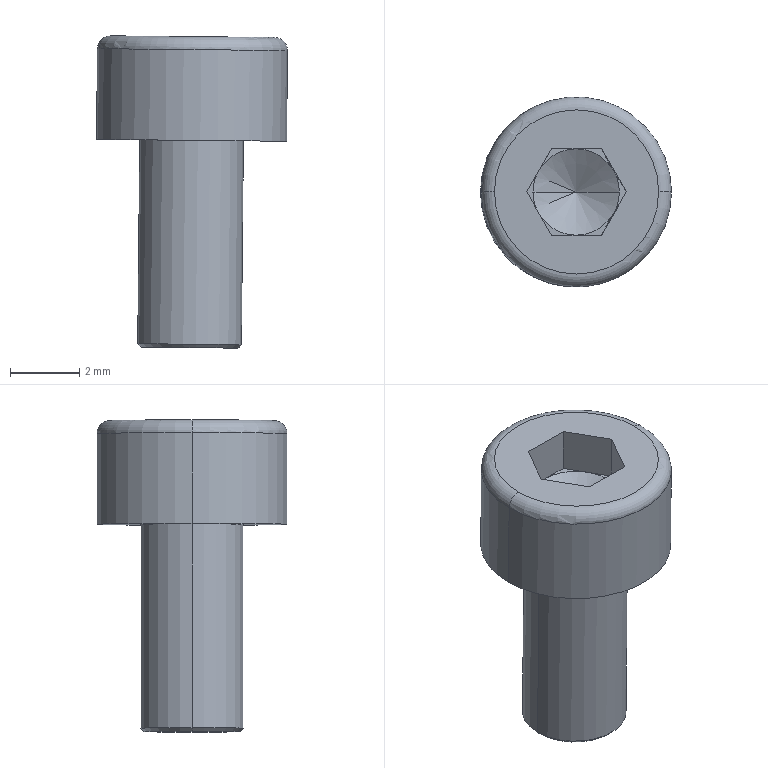Component | SolidWorks | hexagon socket head cap screws gb-20 | 1 solid | 25 faces | box 5.53 x 5.5 x 9.04 mm | volume 105 mm3 | plane 15 | cone 4 | cylinder 4 | torus 2 | commonest cylinder face diameters 3 x2 5.5 x2
STEP:
#1=CARTESIAN_POINT('',(-0.2262,1.201,0.7367));
#2=VERTEX_POINT('',#1);
#3=CARTESIAN_POINT('',(-0.116,1.201,0.7356));
#4=VERTEX_POINT('',#3);
#5=CARTESIAN_POINT('',(-0.1711,1.201,0.7361));
#6=DIRECTION('',(-0.009793,-0.,-1.));
#7=DIRECTION('',(-1.,0.,0.009793));
#8=AXIS2_PLACEMENT_3D('',#5,#6,#7);
#9=CIRCLE('',#8,0.05512);
#10=EDGE_CURVE('',#2,#4,#9,.T.);
#11=ORIENTED_EDGE('',*,*,#10,.F.);
#12=CARTESIAN_POINT('',(-0.2301,1.201,0.7406));
#13=VERTEX_POINT('',#12);
#14=CARTESIAN_POINT('',(-0.2262,1.201,0.7367));
#15=DIRECTION('',(-0.7001,-0.,0.714));
#16=VECTOR('',#15,39.37);
#17=LINE('',#14,#16);
#18=EDGE_CURVE('',#2,#13,#17,.T.);
#19=ORIENTED_EDGE('',*,*,#18,.T.);
#20=CARTESIAN_POINT('',(-0.112,1.201,0.7395));
#21=VERTEX_POINT('',#20);
#22=CARTESIAN_POINT('',(-0.1711,1.201,0.7401));
#23=DIRECTION('',(0.009793,0.,1.));
#24=DIRECTION('',(-1.,-0.,0.009793));
#25=AXIS2_PLACEMENT_3D('',#22,#23,#24);
#26=CIRCLE('',#25,0.05906);
#27=EDGE_CURVE('',#21,#13,#26,.T.);
#28=ORIENTED_EDGE('',*,*,#27,.F.);
#29=CARTESIAN_POINT('',(-0.116,1.201,0.7356));
#30=DIRECTION('',(0.714,0.,0.7001));
#31=VECTOR('',#30,39.37);
#32=LINE('',#29,#31);
#33=EDGE_CURVE('',#4,#21,#32,.T.);
#34=ORIENTED_EDGE('',*,*,#33,.F.);
#35=EDGE_LOOP('',(#11,#19,#28,#34));
#36=FACE_OUTER_BOUND('',#35,.T.);
#37=CARTESIAN_POINT('',(-0.1711,1.201,0.7361));
#38=DIRECTION('',(0.009793,0.,1.));
#39=DIRECTION('',(1.,0.,-0.009793));
#40=AXIS2_PLACEMENT_3D('',#37,#38,#39);
#41=CONICAL_SURFACE('',#40,0.05512,0.7854);
#42=ADVANCED_FACE('',(#36),#41,.T.);
#43=CARTESIAN_POINT('',(-0.07416,1.201,1.09));
#44=VERTEX_POINT('',#43);
#45=CARTESIAN_POINT('',(-0.2612,1.201,1.091));
#46=VERTEX_POINT('',#45);
#47=CARTESIAN_POINT('',(-0.1677,1.201,1.09));
#48=DIRECTION('',(0.009793,0.,1.));
#49=DIRECTION('',(-1.,-0.,0.009793));
#50=AXIS2_PLACEMENT_3D('',#47,#48,#49);
#51=CIRCLE('',#50,0.0935);
#52=EDGE_CURVE('',#44,#46,#51,.T.);
#53=ORIENTED_EDGE('',*,*,#52,.F.);
#54=CARTESIAN_POINT('',(-0.05955,1.201,1.075));
#55=VERTEX_POINT('',#54);
#56=CARTESIAN_POINT('',(-0.07431,1.201,1.075));
#57=DIRECTION('',(-0.,1.,-0.));
#58=DIRECTION('',(-1.,0.,0.));
#59=AXIS2_PLACEMENT_3D('',#56,#57,#58);
#60=CIRCLE('',#59,0.01476);
#61=EDGE_CURVE('',#44,#55,#60,.T.);
#62=ORIENTED_EDGE('',*,*,#61,.T.);
#63=CARTESIAN_POINT('',(-0.2761,1.201,1.077));
#64=VERTEX_POINT('',#63);
#65=CARTESIAN_POINT('',(-0.1678,1.201,1.076));
#66=DIRECTION('',(-0.009793,-0.,-1.));
#67=DIRECTION('',(-1.,-0.,0.009793));
#68=AXIS2_PLACEMENT_3D('',#65,#66,#67);
#69=CIRCLE('',#68,0.1083);
#70=EDGE_CURVE('',#64,#55,#69,.T.);
#71=ORIENTED_EDGE('',*,*,#70,.F.);
#72=CARTESIAN_POINT('',(-0.2613,1.201,1.077));
#73=DIRECTION('',(0.,-1.,0.));
#74=DIRECTION('',(1.,0.,0.));
#75=AXIS2_PLACEMENT_3D('',#72,#73,#74);
#76=CIRCLE('',#75,0.01476);
#77=EDGE_CURVE('',#46,#64,#76,.T.);
#78=ORIENTED_EDGE('',*,*,#77,.F.);
#79=EDGE_LOOP('',(#53,#62,#71,#78));
#80=FACE_OUTER_BOUND('',#79,.T.);
#81=CARTESIAN_POINT('',(-0.1678,1.201,1.076));
#82=DIRECTION('',(-0.009793,-0.,-1.));
#83=DIRECTION('',(-1.,-0.,0.009793));
#84=AXIS2_PLACEMENT_3D('',#81,#82,#83);
#85=TOROIDAL_SURFACE('',#84,0.0935,0.01476);
#86=ADVANCED_FACE('',(#80),#85,.T.);
#87=CARTESIAN_POINT('',(-0.1684,1.201,1.011));
#88=VERTEX_POINT('',#87);
#89=CARTESIAN_POINT('',(-0.119,1.201,1.039));
#90=VERTEX_POINT('',#89);
#91=CARTESIAN_POINT('',(-0.119,1.201,1.039));
#92=DIRECTION('',(0.8709,0.,0.4915));
#93=VECTOR('',#92,39.37);
#94=LINE('',#91,#93);
#95=EDGE_CURVE('',#88,#90,#94,.T.);
#96=ORIENTED_EDGE('',*,*,#95,.F.);
#97=CARTESIAN_POINT('',(-0.2174,1.201,1.04));
#98=VERTEX_POINT('',#97);
#99=CARTESIAN_POINT('',(-0.2174,1.201,1.04));
#100=DIRECTION('',(-0.8611,-0.,0.5085));
#101=VECTOR('',#100,39.37);
#102=LINE('',#99,#101);
#103=EDGE_CURVE('',#88,#98,#102,.T.);
#104=ORIENTED_EDGE('',*,*,#103,.T.);
#105=CARTESIAN_POINT('',(-0.2108,1.176,1.04));
#106=VERTEX_POINT('',#105);
#107=CARTESIAN_POINT('',(-0.1682,1.201,1.039));
#108=DIRECTION('',(-0.009793,-0.,-1.));
#109=DIRECTION('',(1.,0.,-0.009793));
#110=AXIS2_PLACEMENT_3D('',#107,#108,#109);
#111=CIRCLE('',#110,0.04921);
#112=EDGE_CURVE('',#106,#98,#111,.T.);
#113=ORIENTED_EDGE('',*,*,#112,.F.);
#114=CARTESIAN_POINT('',(-0.1682,1.151,1.039));
#115=VERTEX_POINT('',#114);
#116=CARTESIAN_POINT('',(-0.1682,1.201,1.039));
#117=DIRECTION('',(-0.009793,-0.,-1.));
#118=DIRECTION('',(1.,0.,-0.009793));
#119=AXIS2_PLACEMENT_3D('',#116,#117,#118);
#120=CIRCLE('',#119,0.04921);
#121=EDGE_CURVE('',#115,#106,#120,.T.);
#122=ORIENTED_EDGE('',*,*,#121,.F.);
#123=CARTESIAN_POINT('',(-0.1255,1.176,1.039));
#124=VERTEX_POINT('',#123);
#125=CARTESIAN_POINT('',(-0.1682,1.201,1.039));
#126=DIRECTION('',(-0.009793,-0.,-1.));
#127=DIRECTION('',(1.,0.,-0.009793));
#128=AXIS2_PLACEMENT_3D('',#125,#126,#127);
#129=CIRCLE('',#128,0.04921);
#130=EDGE_CURVE('',#124,#115,#129,.T.);
#131=ORIENTED_EDGE('',*,*,#130,.F.);
#132=CARTESIAN_POINT('',(-0.1682,1.201,1.039));
#133=DIRECTION('',(-0.009793,-0.,-1.));
#134=DIRECTION('',(1.,0.,-0.009793));
#135=AXIS2_PLACEMENT_3D('',#132,#133,#134);
#136=CIRCLE('',#135,0.04921);
#137=EDGE_CURVE('',#90,#124,#136,.T.);
#138=ORIENTED_EDGE('',*,*,#137,.F.);
#139=EDGE_LOOP('',(#96,#104,#113,#122,#131,#138));
#140=FACE_OUTER_BOUND('',#139,.T.);
#141=CARTESIAN_POINT('',(-0.1682,1.201,1.039));
#142=DIRECTION('',(0.009793,0.,1.));
#143=DIRECTION('',(1.,0.,-0.009793));
#144=AXIS2_PLACEMENT_3D('',#141,#142,#143);
#145=CONICAL_SURFACE('',#144,0.04921,1.047);
#146=ADVANCED_FACE('',(#140),#145,.F.);
#147=ORIENTED_EDGE('',*,*,#27,.T.);
#148=CARTESIAN_POINT('',(-0.2279,1.201,0.9729));
#149=VERTEX_POINT('',#148);
#150=CARTESIAN_POINT('',(-0.2302,1.201,0.7367));
#151=DIRECTION('',(0.009793,0.,1.));
#152=VECTOR('',#151,39.37);
#153=LINE('',#150,#152);
#154=EDGE_CURVE('',#13,#149,#153,.T.);
#155=ORIENTED_EDGE('',*,*,#154,.T.);
#156=CARTESIAN_POINT('',(-0.1098,1.201,0.9718));
#157=VERTEX_POINT('',#156);
#158=CARTESIAN_POINT('',(-0.1688,1.201,0.9723));
#159=DIRECTION('',(-0.009793,-0.,-1.));
#160=DIRECTION('',(-1.,0.,0.009793));
#161=AXIS2_PLACEMENT_3D('',#158,#159,#160);
#162=CIRCLE('',#161,0.05906);
#163=EDGE_CURVE('',#149,#157,#162,.T.);
#164=ORIENTED_EDGE('',*,*,#163,.T.);
#165=CARTESIAN_POINT('',(-0.1121,1.201,0.7355));
#166=DIRECTION('',(0.009793,0.,1.));
#167=VECTOR('',#166,39.37);
#168=LINE('',#165,#167);
#169=EDGE_CURVE('',#21,#157,#168,.T.);
#170=ORIENTED_EDGE('',*,*,#169,.F.);
#171=EDGE_LOOP('',(#147,#155,#164,#170));
#172=FACE_OUTER_BOUND('',#171,.T.);
#173=CARTESIAN_POINT('',(-0.1711,1.201,0.7361));
#174=DIRECTION('',(0.009793,0.,1.));
#175=DIRECTION('',(1.,0.,-0.009793));
#176=AXIS2_PLACEMENT_3D('',#173,#174,#175);
#177=CYLINDRICAL_SURFACE('',#176,0.05906);
#178=ADVANCED_FACE('',(#172),#177,.T.);
#179=CARTESIAN_POINT('',(-0.2771,1.201,0.9734));
#180=VERTEX_POINT('',#179);
#181=CARTESIAN_POINT('',(-0.06056,1.201,0.9713));
#182=VERTEX_POINT('',#181);
#183=CARTESIAN_POINT('',(-0.1688,1.201,0.9723));
#184=DIRECTION('',(-0.009793,-0.,-1.));
#185=DIRECTION('',(-1.,-0.,0.009793));
#186=AXIS2_PLACEMENT_3D('',#183,#184,#185);
#187=CIRCLE('',#186,0.1083);
#188=EDGE_CURVE('',#180,#182,#187,.T.);
#189=ORIENTED_EDGE('',*,*,#188,.F.);
#190=CARTESIAN_POINT('',(-0.2771,1.201,0.9734));
#191=DIRECTION('',(0.009793,0.,1.));
#192=VECTOR('',#191,39.37);
#193=LINE('',#190,#192);
#194=EDGE_CURVE('',#180,#64,#193,.T.);
#195=ORIENTED_EDGE('',*,*,#194,.T.);
#196=ORIENTED_EDGE('',*,*,#70,.T.);
#197=CARTESIAN_POINT('',(-0.06056,1.201,0.9713));
#198=DIRECTION('',(0.009793,0.,1.));
#199=VECTOR('',#198,39.37);
#200=LINE('',#197,#199);
#201=EDGE_CURVE('',#182,#55,#200,.T.);
#202=ORIENTED_EDGE('',*,*,#201,.F.);
#203=EDGE_LOOP('',(#189,#195,#196,#202));
#204=FACE_OUTER_BOUND('',#203,.T.);
#205=CARTESIAN_POINT('',(-0.1688,1.201,0.9723));
#206=DIRECTION('',(0.009793,0.,1.));
#207=DIRECTION('',(1.,0.,-0.009793));
#208=AXIS2_PLACEMENT_3D('',#205,#206,#207);
#209=CYLINDRICAL_SURFACE('',#208,0.1083);
#210=ADVANCED_FACE('',(#204),#209,.T.);
#211=CARTESIAN_POINT('',(-0.1398,1.151,1.039));
#212=VERTEX_POINT('',#211);
#213=CARTESIAN_POINT('',(-0.1113,1.201,1.039));
#214=DIRECTION('',(-0.5,-0.866,0.004897));
#215=VECTOR('',#214,39.37);
#216=LINE('',#213,#215);
#217=EDGE_CURVE('',#124,#212,#216,.T.);
#218=ORIENTED_EDGE('',*,*,#217,.F.);
#219=ORIENTED_EDGE('',*,*,#130,.T.);
#220=CARTESIAN_POINT('',(-0.1398,1.151,1.039));
#221=DIRECTION('',(-1.,-0.,0.009793));
#222=VECTOR('',#221,39.37);
#223=LINE('',#220,#222);
#224=EDGE_CURVE('',#212,#115,#223,.T.);
#225=ORIENTED_EDGE('',*,*,#224,.F.);
#226=EDGE_LOOP('',(#218,#219,#225));
#227=FACE_OUTER_BOUND('',#226,.T.);
#228=CARTESIAN_POINT('',(-0.1682,1.102,1.039));
#229=DIRECTION('',(0.009793,0.,1.));
#230=DIRECTION('',(1.,0.,-0.009793));
#231=AXIS2_PLACEMENT_3D('',#228,#229,#230);
#232=PLANE('',#231);
#233=ADVANCED_FACE('',(#227),#232,.T.);
#234=CARTESIAN_POINT('',(-0.1966,1.151,1.04));
#235=VERTEX_POINT('',#234);
#236=CARTESIAN_POINT('',(-0.1398,1.151,1.039));
#237=DIRECTION('',(-1.,-0.,0.009793));
#238=VECTOR('',#237,39.37);
#239=LINE('',#236,#238);
#240=EDGE_CURVE('',#115,#235,#239,.T.);
#241=ORIENTED_EDGE('',*,*,#240,.F.);
#242=ORIENTED_EDGE('',*,*,#121,.T.);
#243=CARTESIAN_POINT('',(-0.1966,1.151,1.04));
#244=DIRECTION('',(-0.5,0.866,0.004897));
#245=VECTOR('',#244,39.37);
#246=LINE('',#243,#245);
#247=EDGE_CURVE('',#235,#106,#246,.T.);
#248=ORIENTED_EDGE('',*,*,#247,.F.);
#249=EDGE_LOOP('',(#241,#242,#248));
#250=FACE_OUTER_BOUND('',#249,.T.);
#251=CARTESIAN_POINT('',(-0.1682,1.102,1.039));
#252=DIRECTION('',(0.009793,0.,1.));
#253=DIRECTION('',(1.,0.,-0.009793));
#254=AXIS2_PLACEMENT_3D('',#251,#252,#253);
#255=PLANE('',#254);
#256=ADVANCED_FACE('',(#250),#255,.T.);
#257=CARTESIAN_POINT('',(-0.225,1.201,1.04));
#258=VERTEX_POINT('',#257);
#259=CARTESIAN_POINT('',(-0.1966,1.151,1.04));
#260=DIRECTION('',(-0.5,0.866,0.004897));
#261=VECTOR('',#260,39.37);
#262=LINE('',#259,#261);
#263=EDGE_CURVE('',#106,#258,#262,.T.);
#264=ORIENTED_EDGE('',*,*,#263,.F.);
#265=ORIENTED_EDGE('',*,*,#112,.T.);
#266=CARTESIAN_POINT('',(-0.2108,1.225,1.04));
#267=VERTEX_POINT('',#266);
#268=CARTESIAN_POINT('',(-0.1682,1.201,1.039));
#269=DIRECTION('',(-0.009793,-0.,-1.));
#270=DIRECTION('',(1.,-0.,-0.009793));
#271=AXIS2_PLACEMENT_3D('',#268,#269,#270);
#272=CIRCLE('',#271,0.04921);
#273=EDGE_CURVE('',#98,#267,#272,.T.);
#274=ORIENTED_EDGE('',*,*,#273,.T.);
#275=CARTESIAN_POINT('',(-0.225,1.201,1.04));
#276=DIRECTION('',(0.5,0.866,-0.004897));
#277=VECTOR('',#276,39.37);
#278=LINE('',#275,#277);
#279=EDGE_CURVE('',#258,#267,#278,.T.);
#280=ORIENTED_EDGE('',*,*,#279,.F.);
#281=EDGE_LOOP('',(#264,#265,#274,#280));
#282=FACE_OUTER_BOUND('',#281,.T.);
#283=CARTESIAN_POINT('',(-0.1682,1.102,1.039));
#284=DIRECTION('',(0.009793,0.,1.));
#285=DIRECTION('',(1.,0.,-0.009793));
#286=AXIS2_PLACEMENT_3D('',#283,#284,#285);
#287=PLANE('',#286);
#288=ADVANCED_FACE('',(#282),#287,.T.);
#289=CARTESIAN_POINT('',(-0.1966,1.25,1.04));
#290=VERTEX_POINT('',#289);
#291=CARTESIAN_POINT('',(-0.225,1.201,1.04));
#292=DIRECTION('',(0.5,0.866,-0.004897));
#293=VECTOR('',#292,39.37);
#294=LINE('',#291,#293);
#295=EDGE_CURVE('',#267,#290,#294,.T.);
#296=ORIENTED_EDGE('',*,*,#295,.F.);
#297=CARTESIAN_POINT('',(-0.1682,1.25,1.039));
#298=VERTEX_POINT('',#297);
#299=CARTESIAN_POINT('',(-0.1682,1.201,1.039));
#300=DIRECTION('',(-0.009793,-0.,-1.));
#301=DIRECTION('',(-1.,0.,0.009793));
#302=AXIS2_PLACEMENT_3D('',#299,#300,#301);
#303=CIRCLE('',#302,0.04921);
#304=EDGE_CURVE('',#267,#298,#303,.T.);
#305=ORIENTED_EDGE('',*,*,#304,.T.);
#306=CARTESIAN_POINT('',(-0.1966,1.25,1.04));
#307=DIRECTION('',(1.,0.,-0.009793));
#308=VECTOR('',#307,39.37);
#309=LINE('',#306,#308);
#310=EDGE_CURVE('',#290,#298,#309,.T.);
#311=ORIENTED_EDGE('',*,*,#310,.F.);
#312=EDGE_LOOP('',(#296,#305,#311));
#313=FACE_OUTER_BOUND('',#312,.T.);
#314=CARTESIAN_POINT('',(-0.1682,1.102,1.039));
#315=DIRECTION('',(0.009793,0.,1.));
#316=DIRECTION('',(1.,0.,-0.009793));
#317=AXIS2_PLACEMENT_3D('',#314,#315,#316);
#318=PLANE('',#317);
#319=ADVANCED_FACE('',(#313),#318,.T.);
#320=CARTESIAN_POINT('',(-0.1398,1.25,1.039));
#321=VERTEX_POINT('',#320);
#322=CARTESIAN_POINT('',(-0.1966,1.25,1.04));
#323=DIRECTION('',(1.,0.,-0.009793));
#324=VECTOR('',#323,39.37);
#325=LINE('',#322,#324);
#326=EDGE_CURVE('',#298,#321,#325,.T.);
#327=ORIENTED_EDGE('',*,*,#326,.F.);
#328=CARTESIAN_POINT('',(-0.1255,1.225,1.039));
#329=VERTEX_POINT('',#328);
#330=CARTESIAN_POINT('',(-0.1682,1.201,1.039));
#331=DIRECTION('',(-0.009793,-0.,-1.));
#332=DIRECTION('',(1.,0.,-0.009793));
#333=AXIS2_PLACEMENT_3D('',#330,#331,#332);
#334=CIRCLE('',#333,0.04921);
#335=EDGE_CURVE('',#298,#329,#334,.T.);
#336=ORIENTED_EDGE('',*,*,#335,.T.);
#337=CARTESIAN_POINT('',(-0.1398,1.25,1.039));
#338=DIRECTION('',(0.5,-0.866,-0.004897));
#339=VECTOR('',#338,39.37);
#340=LINE('',#337,#339);
#341=EDGE_CURVE('',#321,#329,#340,.T.);
#342=ORIENTED_EDGE('',*,*,#341,.F.);
#343=EDGE_LOOP('',(#327,#336,#342));
#344=FACE_OUTER_BOUND('',#343,.T.);
#345=CARTESIAN_POINT('',(-0.1682,1.102,1.039));
#346=DIRECTION('',(0.009793,0.,1.));
#347=DIRECTION('',(1.,0.,-0.009793));
#348=AXIS2_PLACEMENT_3D('',#345,#346,#347);
#349=PLANE('',#348);
#350=ADVANCED_FACE('',(#344),#349,.T.);
#351=CARTESIAN_POINT('',(-0.1113,1.201,1.039));
#352=VERTEX_POINT('',#351);
#353=CARTESIAN_POINT('',(-0.1398,1.25,1.039));
#354=DIRECTION('',(0.5,-0.866,-0.004897));
#355=VECTOR('',#354,39.37);
#356=LINE('',#353,#355);
#357=EDGE_CURVE('',#329,#352,#356,.T.);
#358=ORIENTED_EDGE('',*,*,#357,.F.);
#359=CARTESIAN_POINT('',(-0.1682,1.201,1.039));
#360=DIRECTION('',(-0.009793,-0.,-1.));
#361=DIRECTION('',(1.,0.,-0.009793));
#362=AXIS2_PLACEMENT_3D('',#359,#360,#361);
#363=CIRCLE('',#362,0.04921);
#364=EDGE_CURVE('',#329,#90,#363,.T.);
#365=ORIENTED_EDGE('',*,*,#364,.T.);
#366=ORIENTED_EDGE('',*,*,#137,.T.);
#367=CARTESIAN_POINT('',(-0.1113,1.201,1.039));
#368=DIRECTION('',(-0.5,-0.866,0.004897));
#369=VECTOR('',#368,39.37);
#370=LINE('',#367,#369);
#371=EDGE_CURVE('',#352,#124,#370,.T.);
#372=ORIENTED_EDGE('',*,*,#371,.F.);
#373=EDGE_LOOP('',(#358,#365,#366,#372));
#374=FACE_OUTER_BOUND('',#373,.T.);
#375=CARTESIAN_POINT('',(-0.1682,1.102,1.039));
#376=DIRECTION('',(0.009793,0.,1.));
#377=DIRECTION('',(1.,0.,-0.009793));
#378=AXIS2_PLACEMENT_3D('',#375,#376,#377);
#379=PLANE('',#378);
#380=ADVANCED_FACE('',(#374),#379,.T.);
#381=CARTESIAN_POINT('',(-0.1677,1.201,1.09));
#382=DIRECTION('',(0.009793,0.,1.));
#383=DIRECTION('',(-1.,-0.,0.009793));
#384=AXIS2_PLACEMENT_3D('',#381,#382,#383);
#385=CIRCLE('',#384,0.0935);
#386=EDGE_CURVE('',#46,#44,#385,.T.);
#387=ORIENTED_EDGE('',*,*,#386,.T.);
#388=ORIENTED_EDGE('',*,*,#52,.T.);
#389=EDGE_LOOP('',(#387,#388));
#390=FACE_OUTER_BOUND('',#389,.T.);
#391=CARTESIAN_POINT('',(-0.1961,1.151,1.091));
#392=VERTEX_POINT('',#391);
#393=CARTESIAN_POINT('',(-0.2245,1.201,1.091));
#394=VERTEX_POINT('',#393);
#395=CARTESIAN_POINT('',(-0.1961,1.151,1.091));
#396=DIRECTION('',(-0.5,0.866,0.004897));
#397=VECTOR('',#396,39.37);
#398=LINE('',#395,#397);
#399=EDGE_CURVE('',#392,#394,#398,.T.);
#400=ORIENTED_EDGE('',*,*,#399,.T.);
#401=CARTESIAN_POINT('',(-0.1961,1.25,1.091));
#402=VERTEX_POINT('',#401);
#403=CARTESIAN_POINT('',(-0.2245,1.201,1.091));
#404=DIRECTION('',(0.5,0.866,-0.004897));
#405=VECTOR('',#404,39.37);
#406=LINE('',#403,#405);
#407=EDGE_CURVE('',#394,#402,#406,.T.);
#408=ORIENTED_EDGE('',*,*,#407,.T.);
#409=CARTESIAN_POINT('',(-0.1393,1.25,1.09));
#410=VERTEX_POINT('',#409);
#411=CARTESIAN_POINT('',(-0.1961,1.25,1.091));
#412=DIRECTION('',(1.,0.,-0.009793));
#413=VECTOR('',#412,39.37);
#414=LINE('',#411,#413);
#415=EDGE_CURVE('',#402,#410,#414,.T.);
#416=ORIENTED_EDGE('',*,*,#415,.T.);
#417=CARTESIAN_POINT('',(-0.1108,1.201,1.09));
#418=VERTEX_POINT('',#417);
#419=CARTESIAN_POINT('',(-0.1393,1.25,1.09));
#420=DIRECTION('',(0.5,-0.866,-0.004897));
#421=VECTOR('',#420,39.37);
#422=LINE('',#419,#421);
#423=EDGE_CURVE('',#410,#418,#422,.T.);
#424=ORIENTED_EDGE('',*,*,#423,.T.);
#425=CARTESIAN_POINT('',(-0.1393,1.151,1.09));
#426=VERTEX_POINT('',#425);
#427=CARTESIAN_POINT('',(-0.1108,1.201,1.09));
#428=DIRECTION('',(-0.5,-0.866,0.004897));
#429=VECTOR('',#428,39.37);
#430=LINE('',#427,#429);
#431=EDGE_CURVE('',#418,#426,#430,.T.);
#432=ORIENTED_EDGE('',*,*,#431,.T.);
#433=CARTESIAN_POINT('',(-0.1393,1.151,1.09));
#434=DIRECTION('',(-1.,-0.,0.009793));
#435=VECTOR('',#434,39.37);
#436=LINE('',#433,#435);
#437=EDGE_CURVE('',#426,#392,#436,.T.);
#438=ORIENTED_EDGE('',*,*,#437,.T.);
#439=EDGE_LOOP('',(#400,#408,#416,#424,#432,#438));
#440=FACE_BOUND('',#439,.T.);
#441=CARTESIAN_POINT('',(-0.1677,1.201,1.09));
#442=DIRECTION('',(-0.009793,-0.,-1.));
#443=DIRECTION('',(-1.,-0.,0.009793));
#444=AXIS2_PLACEMENT_3D('',#441,#442,#443);
#445=PLANE('',#444);
#446=ADVANCED_FACE('',(#390,#440),#445,.F.);
#447=CARTESIAN_POINT('',(-0.1688,1.201,0.9723));
#448=DIRECTION('',(-0.009793,-0.,-1.));
#449=DIRECTION('',(-1.,-0.,0.009793));
#450=AXIS2_PLACEMENT_3D('',#447,#448,#449);
#451=CIRCLE('',#450,0.1083);
#452=EDGE_CURVE('',#182,#180,#451,.T.);
#453=ORIENTED_EDGE('',*,*,#452,.T.);
#454=ORIENTED_EDGE('',*,*,#188,.T.);
#455=EDGE_LOOP('',(#453,#454));
#456=FACE_OUTER_BOUND('',#455,.T.);
#457=CARTESIAN_POINT('',(-0.1688,1.201,0.9723));
#458=DIRECTION('',(-0.009793,-0.,-1.));
#459=DIRECTION('',(-1.,0.,0.009793));
#460=AXIS2_PLACEMENT_3D('',#457,#458,#459);
#461=CIRCLE('',#460,0.05906);
#462=EDGE_CURVE('',#157,#149,#461,.T.);
#463=ORIENTED_EDGE('',*,*,#462,.F.);
#464=ORIENTED_EDGE('',*,*,#163,.F.);
#465=EDGE_LOOP('',(#463,#464));
#466=FACE_BOUND('',#465,.T.);
#467=CARTESIAN_POINT('',(-0.1688,1.201,0.9723));
#468=DIRECTION('',(-0.009793,-0.,-1.));
#469=DIRECTION('',(-1.,-0.,0.009793));
#470=AXIS2_PLACEMENT_3D('',#467,#468,#469);
#471=PLANE('',#470);
#472=ADVANCED_FACE('',(#456,#466),#471,.T.);
#473=ORIENTED_EDGE('',*,*,#194,.F.);
#474=ORIENTED_EDGE('',*,*,#452,.F.);
#475=ORIENTED_EDGE('',*,*,#201,.T.);
#476=CARTESIAN_POINT('',(-0.1678,1.201,1.076));
#477=DIRECTION('',(-0.009793,-0.,-1.));
#478=DIRECTION('',(-1.,-0.,0.009793));
#479=AXIS2_PLACEMENT_3D('',#476,#477,#478);
#480=CIRCLE('',#479,0.1083);
#481=EDGE_CURVE('',#55,#64,#480,.T.);
#482=ORIENTED_EDGE('',*,*,#481,.T.);
#483=EDGE_LOOP('',(#473,#474,#475,#482));
#484=FACE_OUTER_BOUND('',#483,.T.);
#485=CARTESIAN_POINT('',(-0.1688,1.201,0.9723));
#486=DIRECTION('',(0.009793,0.,1.));
#487=DIRECTION('',(1.,0.,-0.009793));
#488=AXIS2_PLACEMENT_3D('',#485,#486,#487);
#489=CYLINDRICAL_SURFACE('',#488,0.1083);
#490=ADVANCED_FACE('',(#484),#489,.T.);
#491=ORIENTED_EDGE('',*,*,#154,.F.);
#492=CARTESIAN_POINT('',(-0.1711,1.201,0.7401));
#493=DIRECTION('',(0.009793,0.,1.));
#494=DIRECTION('',(-1.,-0.,0.009793));
#495=AXIS2_PLACEMENT_3D('',#492,#493,#494);
#496=CIRCLE('',#495,0.05906);
#497=EDGE_CURVE('',#13,#21,#496,.T.);
#498=ORIENTED_EDGE('',*,*,#497,.T.);
#499=ORIENTED_EDGE('',*,*,#169,.T.);
#500=ORIENTED_EDGE('',*,*,#462,.T.);
#501=EDGE_LOOP('',(#491,#498,#499,#500));
#502=FACE_OUTER_BOUND('',#501,.T.);
#503=CARTESIAN_POINT('',(-0.1711,1.201,0.7361));
#504=DIRECTION('',(0.009793,0.,1.));
#505=DIRECTION('',(1.,0.,-0.009793));
#506=AXIS2_PLACEMENT_3D('',#503,#504,#505);
#507=CYLINDRICAL_SURFACE('',#506,0.05906);
#508=ADVANCED_FACE('',(#502),#507,.T.);
#509=CARTESIAN_POINT('',(-0.1711,1.201,0.7361));
#510=DIRECTION('',(-0.009793,-0.,-1.));
#511=DIRECTION('',(-1.,0.,0.009793));
#512=AXIS2_PLACEMENT_3D('',#509,#510,#511);
#513=CIRCLE('',#512,0.05512);
#514=EDGE_CURVE('',#4,#2,#513,.T.);
#515=ORIENTED_EDGE('',*,*,#514,.T.);
#516=ORIENTED_EDGE('',*,*,#10,.T.);
#517=EDGE_LOOP('',(#515,#516));
#518=FACE_OUTER_BOUND('',#517,.T.);
#519=CARTESIAN_POINT('',(-0.1711,1.201,0.7361));
#520=DIRECTION('',(-0.009793,-0.,-1.));
#521=DIRECTION('',(-1.,-0.,0.009793));
#522=AXIS2_PLACEMENT_3D('',#519,#520,#521);
#523=PLANE('',#522);
#524=ADVANCED_FACE('',(#518),#523,.T.);
#525=ORIENTED_EDGE('',*,*,#399,.F.);
#526=CARTESIAN_POINT('',(-0.1966,1.151,1.04));
#527=DIRECTION('',(0.009793,0.,1.));
#528=VECTOR('',#527,39.37);
#529=LINE('',#526,#528);
#530=EDGE_CURVE('',#235,#392,#529,.T.);
#531=ORIENTED_EDGE('',*,*,#530,.F.);
#532=ORIENTED_EDGE('',*,*,#247,.T.);
#533=ORIENTED_EDGE('',*,*,#263,.T.);
#534=CARTESIAN_POINT('',(-0.225,1.201,1.04));
#535=DIRECTION('',(0.009793,0.,1.));
#536=VECTOR('',#535,39.37);
#537=LINE('',#534,#536);
#538=EDGE_CURVE('',#258,#394,#537,.T.);
#539=ORIENTED_EDGE('',*,*,#538,.T.);
#540=EDGE_LOOP('',(#525,#531,#532,#533,#539));
#541=FACE_OUTER_BOUND('',#540,.T.);
#542=CARTESIAN_POINT('',(-0.1966,1.151,1.04));
#543=DIRECTION('',(0.866,0.5,-0.008481));
#544=DIRECTION('',(0.5,-0.866,-0.004897));
#545=AXIS2_PLACEMENT_3D('',#542,#543,#544);
#546=PLANE('',#545);
#547=ADVANCED_FACE('',(#541),#546,.T.);
#548=ORIENTED_EDGE('',*,*,#407,.F.);
#549=ORIENTED_EDGE('',*,*,#538,.F.);
#550=ORIENTED_EDGE('',*,*,#279,.T.);
#551=ORIENTED_EDGE('',*,*,#295,.T.);
#552=CARTESIAN_POINT('',(-0.1966,1.25,1.04));
#553=DIRECTION('',(0.009793,0.,1.));
#554=VECTOR('',#553,39.37);
#555=LINE('',#552,#554);
#556=EDGE_CURVE('',#290,#402,#555,.T.);
#557=ORIENTED_EDGE('',*,*,#556,.T.);
#558=EDGE_LOOP('',(#548,#549,#550,#551,#557));
#559=FACE_OUTER_BOUND('',#558,.T.);
#560=CARTESIAN_POINT('',(-0.225,1.201,1.04));
#561=DIRECTION('',(0.866,-0.5,-0.008481));
#562=DIRECTION('',(-0.5,-0.866,0.004897));
#563=AXIS2_PLACEMENT_3D('',#560,#561,#562);
#564=PLANE('',#563);
#565=ADVANCED_FACE('',(#559),#564,.T.);
#566=ORIENTED_EDGE('',*,*,#415,.F.);
#567=ORIENTED_EDGE('',*,*,#556,.F.);
#568=ORIENTED_EDGE('',*,*,#310,.T.);
#569=ORIENTED_EDGE('',*,*,#326,.T.);
#570=CARTESIAN_POINT('',(-0.1398,1.25,1.039));
#571=DIRECTION('',(0.009793,0.,1.));
#572=VECTOR('',#571,39.37);
#573=LINE('',#570,#572);
#574=EDGE_CURVE('',#321,#410,#573,.T.);
#575=ORIENTED_EDGE('',*,*,#574,.T.);
#576=EDGE_LOOP('',(#566,#567,#568,#569,#575));
#577=FACE_OUTER_BOUND('',#576,.T.);
#578=CARTESIAN_POINT('',(-0.1966,1.25,1.04));
#579=DIRECTION('',(0.,-1.,0.));
#580=DIRECTION('',(-1.,-0.,0.009793));
#581=AXIS2_PLACEMENT_3D('',#578,#579,#580);
#582=PLANE('',#581);
#583=ADVANCED_FACE('',(#577),#582,.T.);
#584=ORIENTED_EDGE('',*,*,#423,.F.);
#585=ORIENTED_EDGE('',*,*,#574,.F.);
#586=ORIENTED_EDGE('',*,*,#341,.T.);
#587=ORIENTED_EDGE('',*,*,#357,.T.);
#588=CARTESIAN_POINT('',(-0.1113,1.201,1.039));
#589=DIRECTION('',(0.009793,0.,1.));
#590=VECTOR('',#589,39.37);
#591=LINE('',#588,#590);
#592=EDGE_CURVE('',#352,#418,#591,.T.);
#593=ORIENTED_EDGE('',*,*,#592,.T.);
#594=EDGE_LOOP('',(#584,#585,#586,#587,#593));
#595=FACE_OUTER_BOUND('',#594,.T.);
#596=CARTESIAN_POINT('',(-0.1398,1.25,1.039));
#597=DIRECTION('',(-0.866,-0.5,0.008481));
#598=DIRECTION('',(-0.5,0.866,0.004897));
#599=AXIS2_PLACEMENT_3D('',#596,#597,#598);
#600=PLANE('',#599);
#601=ADVANCED_FACE('',(#595),#600,.T.);
#602=ORIENTED_EDGE('',*,*,#431,.F.);
#603=ORIENTED_EDGE('',*,*,#592,.F.);
#604=ORIENTED_EDGE('',*,*,#371,.T.);
#605=ORIENTED_EDGE('',*,*,#217,.T.);
#606=CARTESIAN_POINT('',(-0.1398,1.151,1.039));
#607=DIRECTION('',(0.009793,0.,1.));
#608=VECTOR('',#607,39.37);
#609=LINE('',#606,#608);
#610=EDGE_CURVE('',#212,#426,#609,.T.);
#611=ORIENTED_EDGE('',*,*,#610,.T.);
#612=EDGE_LOOP('',(#602,#603,#604,#605,#611));
#613=FACE_OUTER_BOUND('',#612,.T.);
#614=CARTESIAN_POINT('',(-0.1113,1.201,1.039));
#615=DIRECTION('',(-0.866,0.5,0.008481));
#616=DIRECTION('',(0.5,0.866,-0.004897));
#617=AXIS2_PLACEMENT_3D('',#614,#615,#616);
#618=PLANE('',#617);
#619=ADVANCED_FACE('',(#613),#618,.T.);
#620=ORIENTED_EDGE('',*,*,#437,.F.);
#621=ORIENTED_EDGE('',*,*,#610,.F.);
#622=ORIENTED_EDGE('',*,*,#224,.T.);
#623=ORIENTED_EDGE('',*,*,#240,.T.);
#624=ORIENTED_EDGE('',*,*,#530,.T.);
#625=EDGE_LOOP('',(#620,#621,#622,#623,#624));
#626=FACE_OUTER_BOUND('',#625,.T.);
#627=CARTESIAN_POINT('',(-0.1398,1.151,1.039));
#628=DIRECTION('',(-0.,1.,-0.));
#629=DIRECTION('',(1.,0.,-0.009793));
#630=AXIS2_PLACEMENT_3D('',#627,#628,#629);
#631=PLANE('',#630);
#632=ADVANCED_FACE('',(#626),#631,.T.);
#633=ORIENTED_EDGE('',*,*,#103,.F.);
#634=ORIENTED_EDGE('',*,*,#95,.T.);
#635=ORIENTED_EDGE('',*,*,#364,.F.);
#636=ORIENTED_EDGE('',*,*,#335,.F.);
#637=ORIENTED_EDGE('',*,*,#304,.F.);
#638=ORIENTED_EDGE('',*,*,#273,.F.);
#639=EDGE_LOOP('',(#633,#634,#635,#636,#637,#638));
#640=FACE_OUTER_BOUND('',#639,.T.);
#641=CARTESIAN_POINT('',(-0.1682,1.201,1.039));
#642=DIRECTION('',(0.009793,0.,1.));
#643=DIRECTION('',(1.,0.,-0.009793));
#644=AXIS2_PLACEMENT_3D('',#641,#642,#643);
#645=CONICAL_SURFACE('',#644,0.04921,1.047);
#646=ADVANCED_FACE('',(#640),#645,.F.);
#647=ORIENTED_EDGE('',*,*,#61,.F.);
#648=ORIENTED_EDGE('',*,*,#386,.F.);
#649=ORIENTED_EDGE('',*,*,#77,.T.);
#650=ORIENTED_EDGE('',*,*,#481,.F.);
#651=EDGE_LOOP('',(#647,#648,#649,#650));
#652=FACE_OUTER_BOUND('',#651,.T.);
#653=CARTESIAN_POINT('',(-0.1678,1.201,1.076));
#654=DIRECTION('',(-0.009793,-0.,-1.));
#655=DIRECTION('',(-1.,-0.,0.009793));
#656=AXIS2_PLACEMENT_3D('',#653,#654,#655);
#657=TOROIDAL_SURFACE('',#656,0.0935,0.01476);
#658=ADVANCED_FACE('',(#652),#657,.T.);
#659=ORIENTED_EDGE('',*,*,#18,.F.);
#660=ORIENTED_EDGE('',*,*,#514,.F.);
#661=ORIENTED_EDGE('',*,*,#33,.T.);
#662=ORIENTED_EDGE('',*,*,#497,.F.);
#663=EDGE_LOOP('',(#659,#660,#661,#662));
#664=FACE_OUTER_BOUND('',#663,.T.);
#665=CARTESIAN_POINT('',(-0.1711,1.201,0.7361));
#666=DIRECTION('',(0.009793,0.,1.));
#667=DIRECTION('',(1.,0.,-0.009793));
#668=AXIS2_PLACEMENT_3D('',#665,#666,#667);
#669=CONICAL_SURFACE('',#668,0.05512,0.7854);
#670=ADVANCED_FACE('',(#664),#669,.T.);
#671=CLOSED_SHELL('',(#42,#86,#146,#178,#210,#233,#256,#288,#319,#350,#380,#446,#472,#490,#508,#524,#547,#565,#583,#601,#619,#632,#646,#658,#670));
#672=MANIFOLD_SOLID_BREP('',#671);
#673=CARTESIAN_POINT('',(0.,0.,0.));
#674=DIRECTION('',(0.,0.,1.));
#675=DIRECTION('',(1.,0.,0.));
#676=AXIS2_PLACEMENT_3D('',#673,#674,#675);
#677=(LENGTH_UNIT()NAMED_UNIT(*)SI_UNIT($,.METRE.));
#678=LENGTH_MEASURE_WITH_UNIT(LENGTH_MEASURE(0.0254),#677);
#679=DIMENSIONAL_EXPONENTS(1.,0.,0.,0.,0.,0.,0.);
#680=(CONVERSION_BASED_UNIT('',#678)LENGTH_UNIT()NAMED_UNIT(#679));
#681=UNCERTAINTY_MEASURE_WITH_UNIT(LENGTH_MEASURE(0.00001),#680,'','');
#682=(NAMED_UNIT(*)PLANE_ANGLE_UNIT()SI_UNIT($,.RADIAN.));
#683=(NAMED_UNIT(*)SI_UNIT($,.STERADIAN.)SOLID_ANGLE_UNIT());
#684=(GEOMETRIC_REPRESENTATION_CONTEXT(3)GLOBAL_UNCERTAINTY_ASSIGNED_CONTEXT((#681))GLOBAL_UNIT_ASSIGNED_CONTEXT((#680,#682,#683))REPRESENTATION_CONTEXT('',''));
#685=ADVANCED_BREP_SHAPE_REPRESENTATION('',(#672,#676),#684);
#686=COLOUR_RGB('',0.7922,0.8196,0.9333);
#687=FILL_AREA_STYLE_COLOUR('',#686);
#688=FILL_AREA_STYLE('',(#687));
#689=SURFACE_STYLE_FILL_AREA(#688);
#690=SURFACE_SIDE_STYLE('',(#689));
#691=SURFACE_STYLE_USAGE(.BOTH.,#690);
#692=PRESENTATION_STYLE_ASSIGNMENT((#691));
#693=STYLED_ITEM('',(#692),#672);
#694=PRESENTATION_LAYER_ASSIGNMENT('','',(#693));
#695=(LENGTH_UNIT()NAMED_UNIT(*)SI_UNIT($,.METRE.));
#696=LENGTH_MEASURE_WITH_UNIT(LENGTH_MEASURE(0.0254),#695);
#697=DIMENSIONAL_EXPONENTS(1.,0.,0.,0.,0.,0.,0.);
#698=(CONVERSION_BASED_UNIT('',#696)LENGTH_UNIT()NAMED_UNIT(#697));
#699=UNCERTAINTY_MEASURE_WITH_UNIT(LENGTH_MEASURE(0.00001),#698,'','');
#700=(NAMED_UNIT(*)PLANE_ANGLE_UNIT()SI_UNIT($,.RADIAN.));
#701=(NAMED_UNIT(*)SI_UNIT($,.STERADIAN.)SOLID_ANGLE_UNIT());
#702=(GEOMETRIC_REPRESENTATION_CONTEXT(3)GLOBAL_UNCERTAINTY_ASSIGNED_CONTEXT((#699))GLOBAL_UNIT_ASSIGNED_CONTEXT((#698,#700,#701))REPRESENTATION_CONTEXT('',''));
#703=MECHANICAL_DESIGN_GEOMETRIC_PRESENTATION_REPRESENTATION('',(#693),#702);